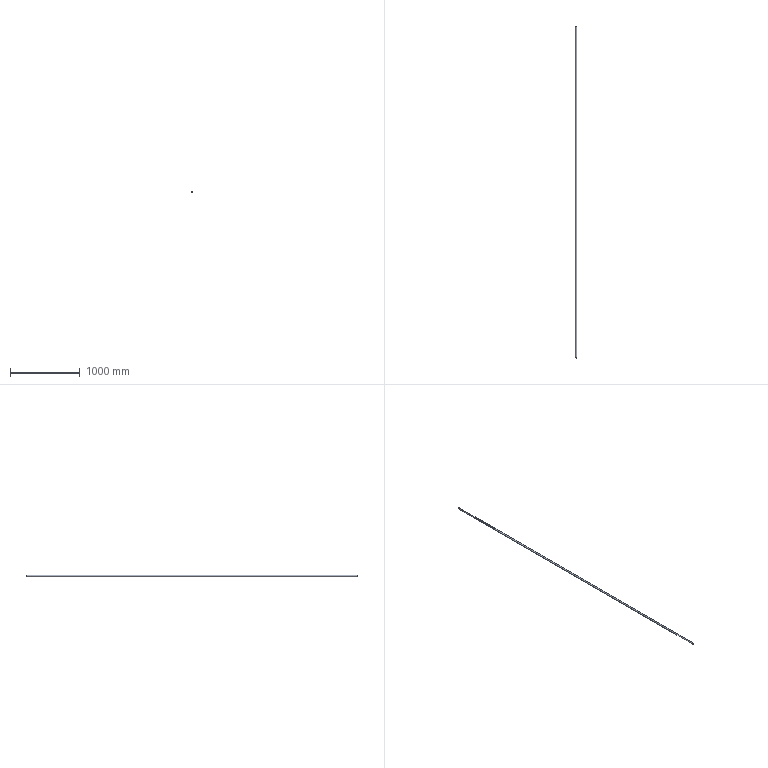Component | NX | 44_2 | 1 solid | 4 faces | volume 537212 mm3 | cylinder 2 | plane 2 | commonest cylinder face diameters 20 x1 16 x1